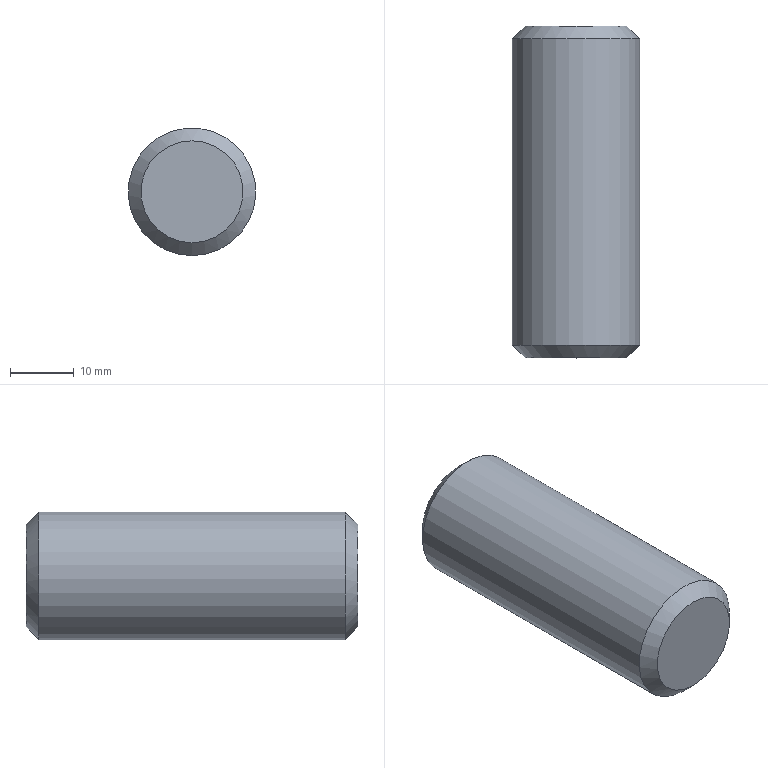Component | NX | PISTON_PIN_2 | 1 solid | 5 faces | box 20 x 52 x 20 mm | volume 16102 mm3 | plane 2 | cone 2 | cylinder 1 | commonest cylinder face diameters 20 x1
STEP:
#1=CARTESIAN_POINT('',(0.,0.,0.));
#2=DIRECTION('',(0.,0.,1.));
#3=DIRECTION('',(1.,0.,0.));
#4=AXIS2_PLACEMENT_3D('',#1,#2,#3);
#5=CARTESIAN_POINT('',(-0.,24.,24.214));
#6=VERTEX_POINT('',#5);
#7=CARTESIAN_POINT('',(-0.,24.,34.214));
#8=DIRECTION('',(0.,-1.,0.));
#9=DIRECTION('',(0.,0.,-1.));
#10=AXIS2_PLACEMENT_3D('',#7,#8,#9);
#11=CIRCLE('',#10,10.);
#12=CARTESIAN_POINT('',(-0.,26.,34.214));
#13=DIRECTION('',(0.,-1.,0.));
#14=DIRECTION('',(0.,0.,-1.));
#15=AXIS2_PLACEMENT_3D('',#12,#13,#14);
#16=CYLINDRICAL_SURFACE('',#15,10.);
#17=CARTESIAN_POINT('',(0.,2.));
#18=DIRECTION('',(1.,0.));
#19=VECTOR('',#18,1.);
#20=LINE('',#17,#19);
#21=(GEOMETRIC_REPRESENTATION_CONTEXT(2)PARAMETRIC_REPRESENTATION_CONTEXT()REPRESENTATION_CONTEXT('',''));
#22=DEFINITIONAL_REPRESENTATION('',(#20),#21);
#23=PCURVE('',#16,#22);
#24=CARTESIAN_POINT('',(-0.,24.,34.214));
#25=DIRECTION('',(0.,-1.,0.));
#26=DIRECTION('',(0.,0.,-1.));
#27=AXIS2_PLACEMENT_3D('',#24,#25,#26);
#28=CONICAL_SURFACE('',#27,10.,0.7854);
#29=CARTESIAN_POINT('',(0.,0.));
#30=DIRECTION('',(1.,0.));
#31=VECTOR('',#30,1.);
#32=LINE('',#29,#31);
#33=(GEOMETRIC_REPRESENTATION_CONTEXT(2)PARAMETRIC_REPRESENTATION_CONTEXT()REPRESENTATION_CONTEXT('',''));
#34=DEFINITIONAL_REPRESENTATION('',(#32),#33);
#35=PCURVE('',#28,#34);
#36=SURFACE_CURVE('',#11,(#23,#35),.PCURVE_S1.);
#37=EDGE_CURVE('',#6,#6,#36,.T.);
#38=ORIENTED_EDGE('',*,*,#37,.T.);
#39=CARTESIAN_POINT('',(-0.,-24.,24.214));
#40=VERTEX_POINT('',#39);
#41=CARTESIAN_POINT('',(-0.,24.,24.214));
#42=CARTESIAN_POINT('',(-0.,-24.,24.214));
#43=B_SPLINE_CURVE_WITH_KNOTS('',1,(#41,#42),.UNSPECIFIED.,.F.,.F.,(2,2),(2.,50.),.PIECEWISE_BEZIER_KNOTS.);
#44=CARTESIAN_POINT('',(6.283,0.));
#45=DIRECTION('',(0.,1.));
#46=VECTOR('',#45,1.);
#47=LINE('',#44,#46);
#48=(GEOMETRIC_REPRESENTATION_CONTEXT(2)PARAMETRIC_REPRESENTATION_CONTEXT()REPRESENTATION_CONTEXT('',''));
#49=DEFINITIONAL_REPRESENTATION('',(#47),#48);
#50=PCURVE('',#16,#49);
#51=CARTESIAN_POINT('',(0.,0.));
#52=DIRECTION('',(0.,1.));
#53=VECTOR('',#52,1.);
#54=LINE('',#51,#53);
#55=(GEOMETRIC_REPRESENTATION_CONTEXT(2)PARAMETRIC_REPRESENTATION_CONTEXT()REPRESENTATION_CONTEXT('',''));
#56=DEFINITIONAL_REPRESENTATION('',(#54),#55);
#57=PCURVE('',#16,#56);
#58=SEAM_CURVE('',#43,(#50,#57),.PCURVE_S1.);
#59=EDGE_CURVE('',#6,#40,#58,.T.);
#60=ORIENTED_EDGE('',*,*,#59,.T.);
#61=CARTESIAN_POINT('',(-0.,-24.,34.214));
#62=DIRECTION('',(0.,1.,0.));
#63=DIRECTION('',(0.,0.,-1.));
#64=AXIS2_PLACEMENT_3D('',#61,#62,#63);
#65=CIRCLE('',#64,10.);
#66=CARTESIAN_POINT('',(6.283,50.));
#67=DIRECTION('',(-1.,0.));
#68=VECTOR('',#67,1.);
#69=LINE('',#66,#68);
#70=(GEOMETRIC_REPRESENTATION_CONTEXT(2)PARAMETRIC_REPRESENTATION_CONTEXT()REPRESENTATION_CONTEXT('',''));
#71=DEFINITIONAL_REPRESENTATION('',(#69),#70);
#72=PCURVE('',#16,#71);
#73=CARTESIAN_POINT('',(-0.,-26.,34.214));
#74=DIRECTION('',(0.,1.,0.));
#75=DIRECTION('',(0.,0.,1.));
#76=AXIS2_PLACEMENT_3D('',#73,#74,#75);
#77=CONICAL_SURFACE('',#76,8.,0.7854);
#78=CARTESIAN_POINT('',(3.142,2.));
#79=DIRECTION('',(1.,0.));
#80=VECTOR('',#79,1.);
#81=LINE('',#78,#80);
#82=(GEOMETRIC_REPRESENTATION_CONTEXT(2)PARAMETRIC_REPRESENTATION_CONTEXT()REPRESENTATION_CONTEXT('',''));
#83=DEFINITIONAL_REPRESENTATION('',(#81),#82);
#84=PCURVE('',#77,#83);
#85=SURFACE_CURVE('',#65,(#72,#84),.PCURVE_S1.);
#86=EDGE_CURVE('',#40,#40,#85,.T.);
#87=ORIENTED_EDGE('',*,*,#86,.T.);
#88=ORIENTED_EDGE('',*,*,#59,.F.);
#89=EDGE_LOOP('',(#38,#60,#87,#88));
#90=FACE_BOUND('',#89,.T.);
#91=ADVANCED_FACE('',(#90),#16,.T.);
#92=CARTESIAN_POINT('',(-0.,26.,26.214));
#93=VERTEX_POINT('',#92);
#94=CARTESIAN_POINT('',(-0.,26.,34.214));
#95=DIRECTION('',(0.,1.,0.));
#96=DIRECTION('',(0.,0.,-1.));
#97=AXIS2_PLACEMENT_3D('',#94,#95,#96);
#98=CIRCLE('',#97,8.);
#99=CARTESIAN_POINT('',(-0.,26.,34.214));
#100=DIRECTION('',(0.,-1.,0.));
#101=DIRECTION('',(0.,0.,-1.));
#102=AXIS2_PLACEMENT_3D('',#99,#100,#101);
#103=PLANE('',#102);
#104=CARTESIAN_POINT('',(8.,0.));
#105=CARTESIAN_POINT('',(8.,-13.856));
#106=CARTESIAN_POINT('',(-4.,-6.928));
#107=CARTESIAN_POINT('',(-16.,-0.));
#108=CARTESIAN_POINT('',(-4.,6.928));
#109=CARTESIAN_POINT('',(8.,13.856));
#110=CARTESIAN_POINT('',(8.,0.));
#111=(BOUNDED_CURVE()B_SPLINE_CURVE(2,(#104,#105,#106,#107,#108,#109,#110),.UNSPECIFIED.,.T.,.F.)B_SPLINE_CURVE_WITH_KNOTS((1,2,2,2,2,1),(-2.094,0.,2.094,4.189,6.283,8.378),.UNSPECIFIED.)CURVE()GEOMETRIC_REPRESENTATION_ITEM()RATIONAL_B_SPLINE_CURVE((1.,0.5,1.,0.5,1.,0.5,1.))REPRESENTATION_ITEM(''));
#112=(GEOMETRIC_REPRESENTATION_CONTEXT(2)PARAMETRIC_REPRESENTATION_CONTEXT()REPRESENTATION_CONTEXT('',''));
#113=DEFINITIONAL_REPRESENTATION('',(#111),#112);
#114=PCURVE('',#103,#113);
#115=CARTESIAN_POINT('',(6.283,-2.));
#116=DIRECTION('',(-1.,0.));
#117=VECTOR('',#116,1.);
#118=LINE('',#115,#117);
#119=(GEOMETRIC_REPRESENTATION_CONTEXT(2)PARAMETRIC_REPRESENTATION_CONTEXT()REPRESENTATION_CONTEXT('',''));
#120=DEFINITIONAL_REPRESENTATION('',(#118),#119);
#121=PCURVE('',#28,#120);
#122=SURFACE_CURVE('',#98,(#114,#121),.PCURVE_S1.);
#123=EDGE_CURVE('',#93,#93,#122,.T.);
#124=ORIENTED_EDGE('',*,*,#123,.T.);
#125=EDGE_LOOP('',(#124));
#126=FACE_BOUND('',#125,.T.);
#127=ADVANCED_FACE('',(#126),#103,.F.);
#128=CARTESIAN_POINT('',(-0.,-26.,26.214));
#129=VERTEX_POINT('',#128);
#130=CARTESIAN_POINT('',(-0.,-26.,34.214));
#131=DIRECTION('',(0.,-1.,0.));
#132=DIRECTION('',(0.,0.,-1.));
#133=AXIS2_PLACEMENT_3D('',#130,#131,#132);
#134=CIRCLE('',#133,8.);
#135=CARTESIAN_POINT('',(-0.,-26.,34.214));
#136=DIRECTION('',(0.,-1.,0.));
#137=DIRECTION('',(0.,0.,-1.));
#138=AXIS2_PLACEMENT_3D('',#135,#136,#137);
#139=PLANE('',#138);
#140=CARTESIAN_POINT('',(0.,0.));
#141=DIRECTION('',(1.,0.));
#142=AXIS2_PLACEMENT_2D('',#140,#141);
#143=CIRCLE('',#142,8.);
#144=(GEOMETRIC_REPRESENTATION_CONTEXT(2)PARAMETRIC_REPRESENTATION_CONTEXT()REPRESENTATION_CONTEXT('',''));
#145=DEFINITIONAL_REPRESENTATION('',(#143),#144);
#146=PCURVE('',#139,#145);
#147=CARTESIAN_POINT('',(9.425,0.));
#148=DIRECTION('',(-1.,0.));
#149=VECTOR('',#148,1.);
#150=LINE('',#147,#149);
#151=(GEOMETRIC_REPRESENTATION_CONTEXT(2)PARAMETRIC_REPRESENTATION_CONTEXT()REPRESENTATION_CONTEXT('',''));
#152=DEFINITIONAL_REPRESENTATION('',(#150),#151);
#153=PCURVE('',#77,#152);
#154=SURFACE_CURVE('',#134,(#146,#153),.PCURVE_S1.);
#155=EDGE_CURVE('',#129,#129,#154,.T.);
#156=ORIENTED_EDGE('',*,*,#155,.T.);
#157=EDGE_LOOP('',(#156));
#158=FACE_BOUND('',#157,.T.);
#159=ADVANCED_FACE('',(#158),#139,.T.);
#160=ORIENTED_EDGE('',*,*,#123,.F.);
#161=CARTESIAN_POINT('',(-0.,26.,26.214));
#162=CARTESIAN_POINT('',(-0.,24.,24.214));
#163=B_SPLINE_CURVE_WITH_KNOTS('',1,(#161,#162),.UNSPECIFIED.,.F.,.F.,(2,2),(-2.828,0.),.PIECEWISE_BEZIER_KNOTS.);
#164=CARTESIAN_POINT('',(6.283,0.));
#165=DIRECTION('',(0.,1.));
#166=VECTOR('',#165,1.);
#167=LINE('',#164,#166);
#168=(GEOMETRIC_REPRESENTATION_CONTEXT(2)PARAMETRIC_REPRESENTATION_CONTEXT()REPRESENTATION_CONTEXT('',''));
#169=DEFINITIONAL_REPRESENTATION('',(#167),#168);
#170=PCURVE('',#28,#169);
#171=CARTESIAN_POINT('',(0.,0.));
#172=DIRECTION('',(0.,1.));
#173=VECTOR('',#172,1.);
#174=LINE('',#171,#173);
#175=(GEOMETRIC_REPRESENTATION_CONTEXT(2)PARAMETRIC_REPRESENTATION_CONTEXT()REPRESENTATION_CONTEXT('',''));
#176=DEFINITIONAL_REPRESENTATION('',(#174),#175);
#177=PCURVE('',#28,#176);
#178=SEAM_CURVE('',#163,(#170,#177),.PCURVE_S1.);
#179=EDGE_CURVE('',#93,#6,#178,.T.);
#180=ORIENTED_EDGE('',*,*,#179,.T.);
#181=ORIENTED_EDGE('',*,*,#37,.F.);
#182=ORIENTED_EDGE('',*,*,#179,.F.);
#183=EDGE_LOOP('',(#160,#180,#181,#182));
#184=FACE_BOUND('',#183,.T.);
#185=ADVANCED_FACE('',(#184),#28,.T.);
#186=ORIENTED_EDGE('',*,*,#86,.F.);
#187=CARTESIAN_POINT('',(-0.,-26.,26.214));
#188=CARTESIAN_POINT('',(-0.,-24.,24.214));
#189=B_SPLINE_CURVE_WITH_KNOTS('',1,(#187,#188),.UNSPECIFIED.,.F.,.F.,(2,2),(0.,2.828),.PIECEWISE_BEZIER_KNOTS.);
#190=CARTESIAN_POINT('',(3.142,0.));
#191=DIRECTION('',(0.,1.));
#192=VECTOR('',#191,1.);
#193=LINE('',#190,#192);
#194=(GEOMETRIC_REPRESENTATION_CONTEXT(2)PARAMETRIC_REPRESENTATION_CONTEXT()REPRESENTATION_CONTEXT('',''));
#195=DEFINITIONAL_REPRESENTATION('',(#193),#194);
#196=PCURVE('',#77,#195);
#197=CARTESIAN_POINT('',(9.425,0.));
#198=DIRECTION('',(0.,1.));
#199=VECTOR('',#198,1.);
#200=LINE('',#197,#199);
#201=(GEOMETRIC_REPRESENTATION_CONTEXT(2)PARAMETRIC_REPRESENTATION_CONTEXT()REPRESENTATION_CONTEXT('',''));
#202=DEFINITIONAL_REPRESENTATION('',(#200),#201);
#203=PCURVE('',#77,#202);
#204=SEAM_CURVE('',#189,(#196,#203),.PCURVE_S1.);
#205=EDGE_CURVE('',#129,#40,#204,.T.);
#206=ORIENTED_EDGE('',*,*,#205,.F.);
#207=ORIENTED_EDGE('',*,*,#155,.F.);
#208=ORIENTED_EDGE('',*,*,#205,.T.);
#209=EDGE_LOOP('',(#186,#206,#207,#208));
#210=FACE_BOUND('',#209,.T.);
#211=ADVANCED_FACE('',(#210),#77,.T.);
#212=CLOSED_SHELL('',(#91,#127,#159,#185,#211));
#213=MANIFOLD_SOLID_BREP('',#212);
#214=(LENGTH_UNIT()NAMED_UNIT(*)SI_UNIT(.MILLI.,.METRE.));
#215=UNCERTAINTY_MEASURE_WITH_UNIT(LENGTH_MEASURE(0.00001),#214,'','');
#216=(NAMED_UNIT(*)PLANE_ANGLE_UNIT()SI_UNIT($,.RADIAN.));
#217=(NAMED_UNIT(*)SI_UNIT($,.STERADIAN.)SOLID_ANGLE_UNIT());
#218=(GEOMETRIC_REPRESENTATION_CONTEXT(3)GLOBAL_UNCERTAINTY_ASSIGNED_CONTEXT((#215))GLOBAL_UNIT_ASSIGNED_CONTEXT((#214,#216,#217))REPRESENTATION_CONTEXT('',''));
#219=ADVANCED_BREP_SHAPE_REPRESENTATION('',(#4,#213),#218);